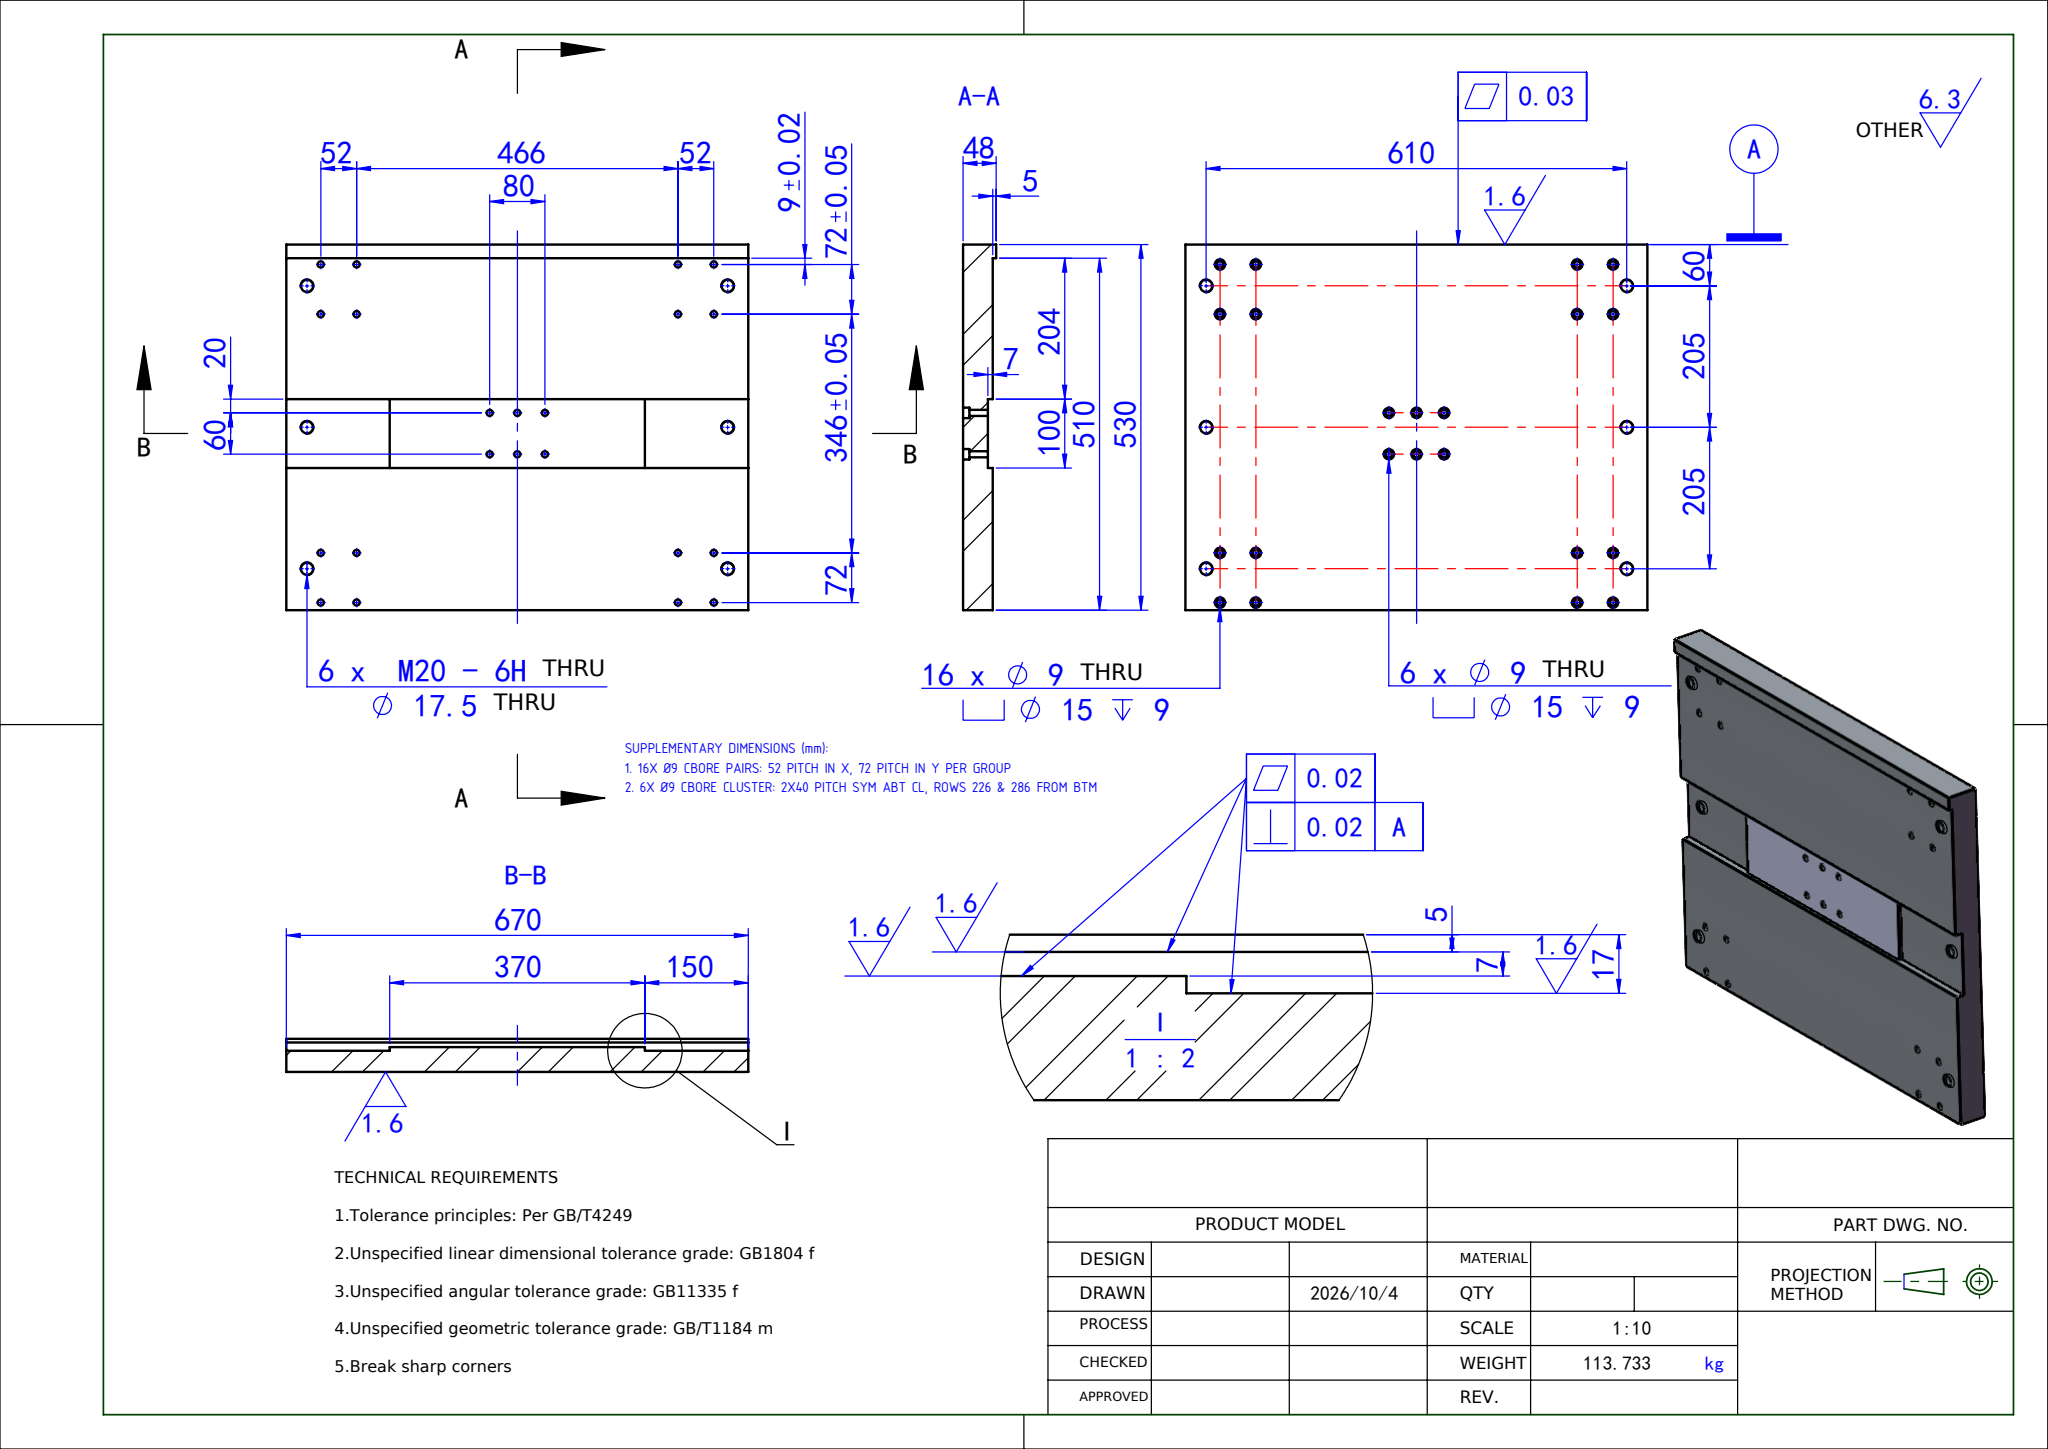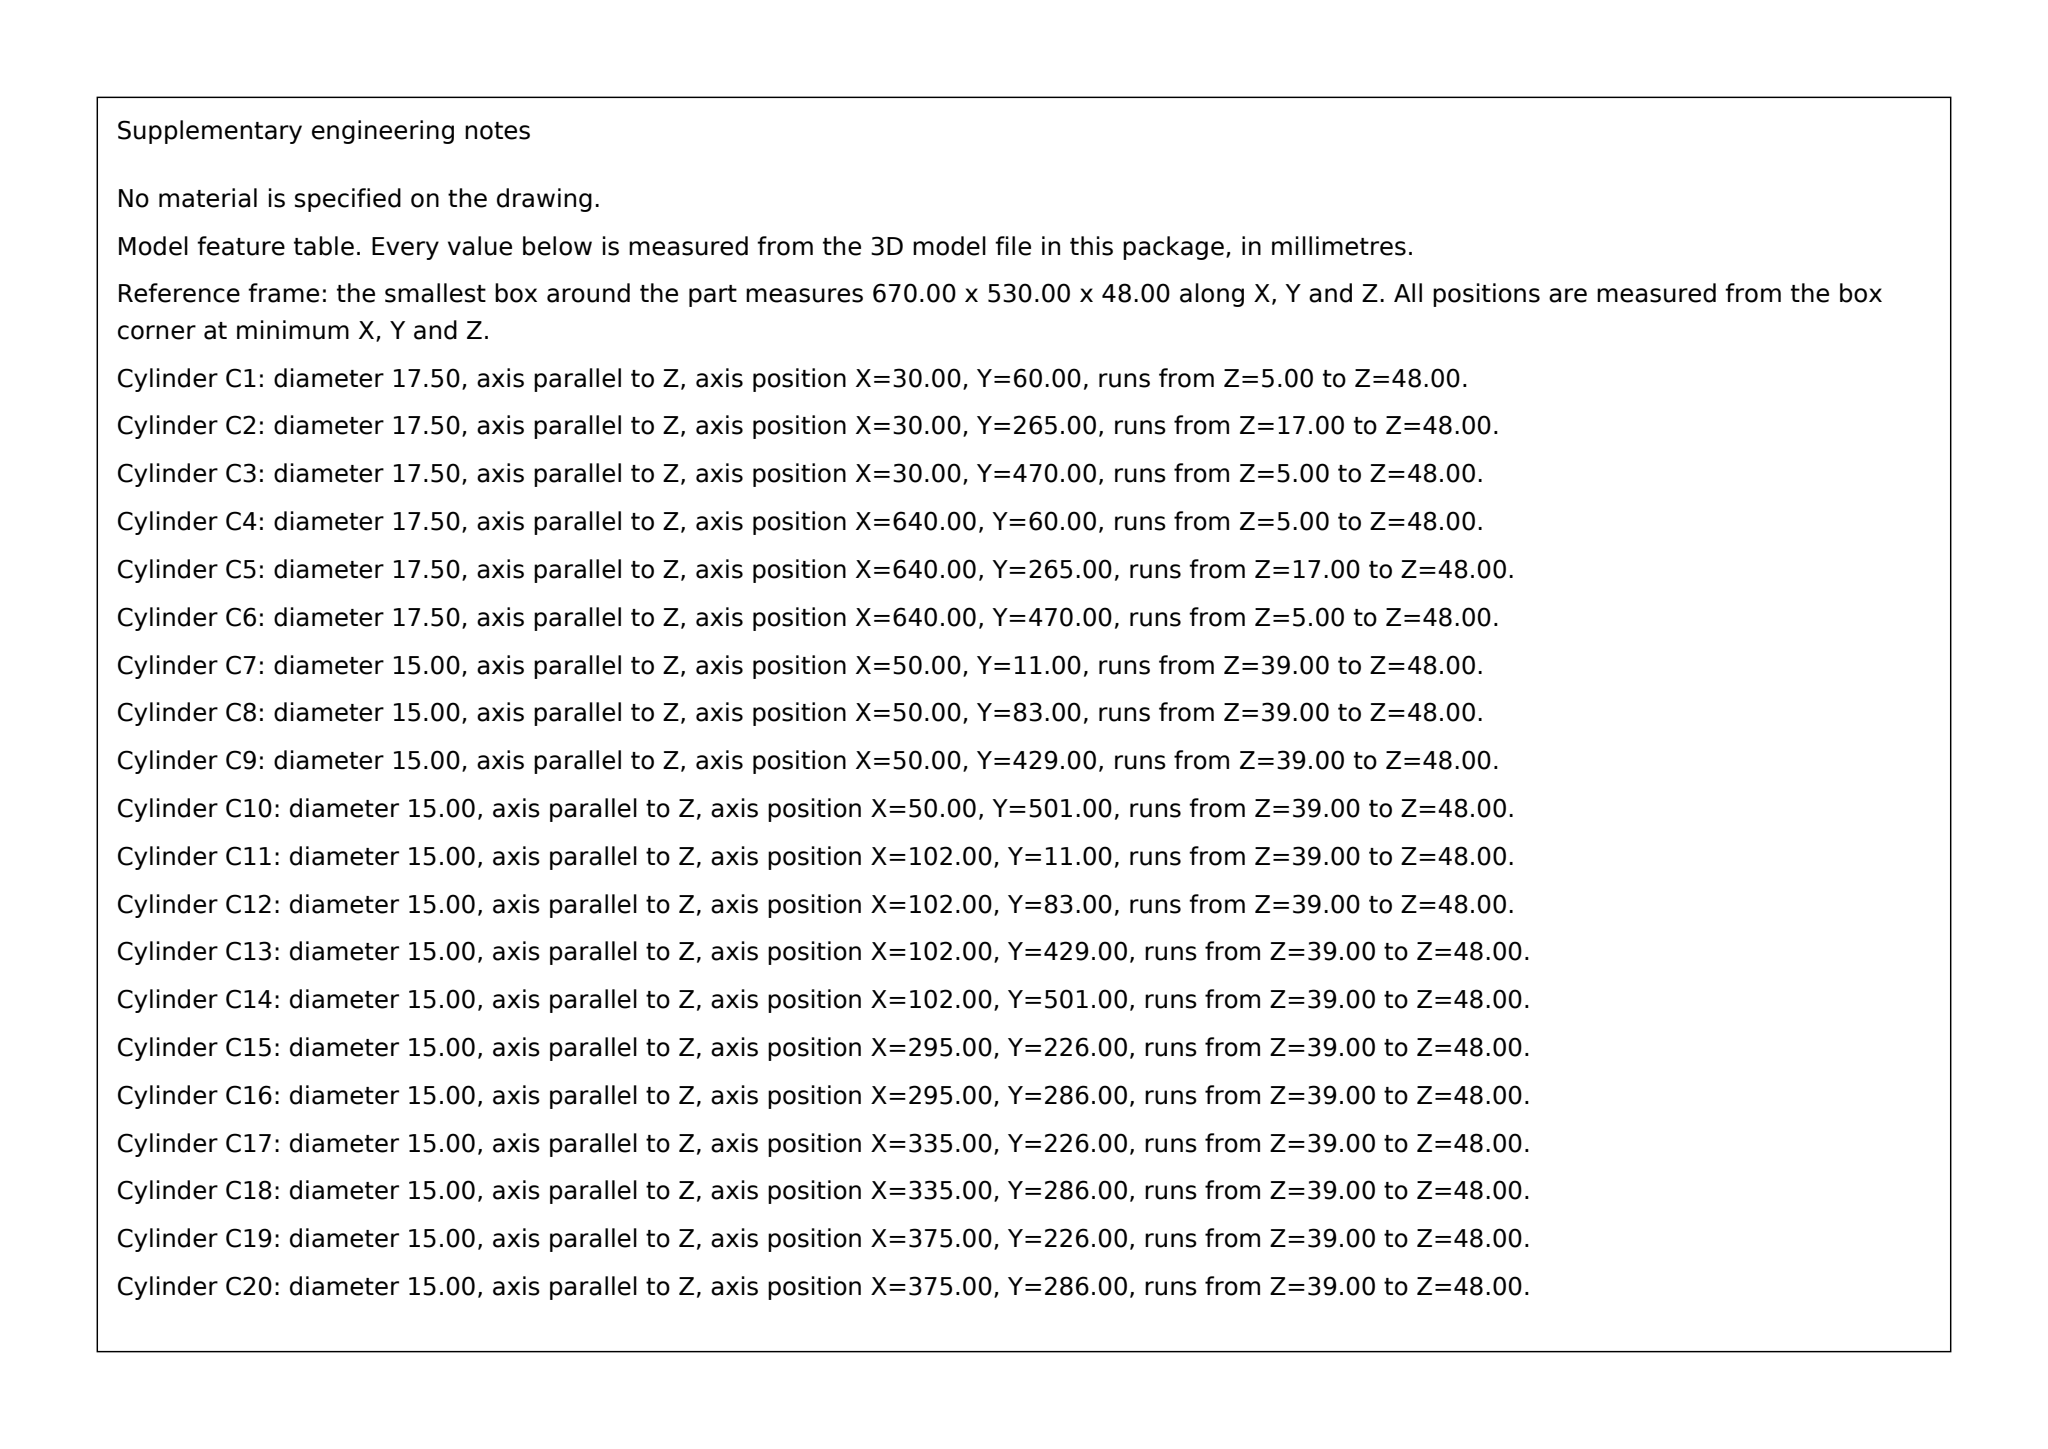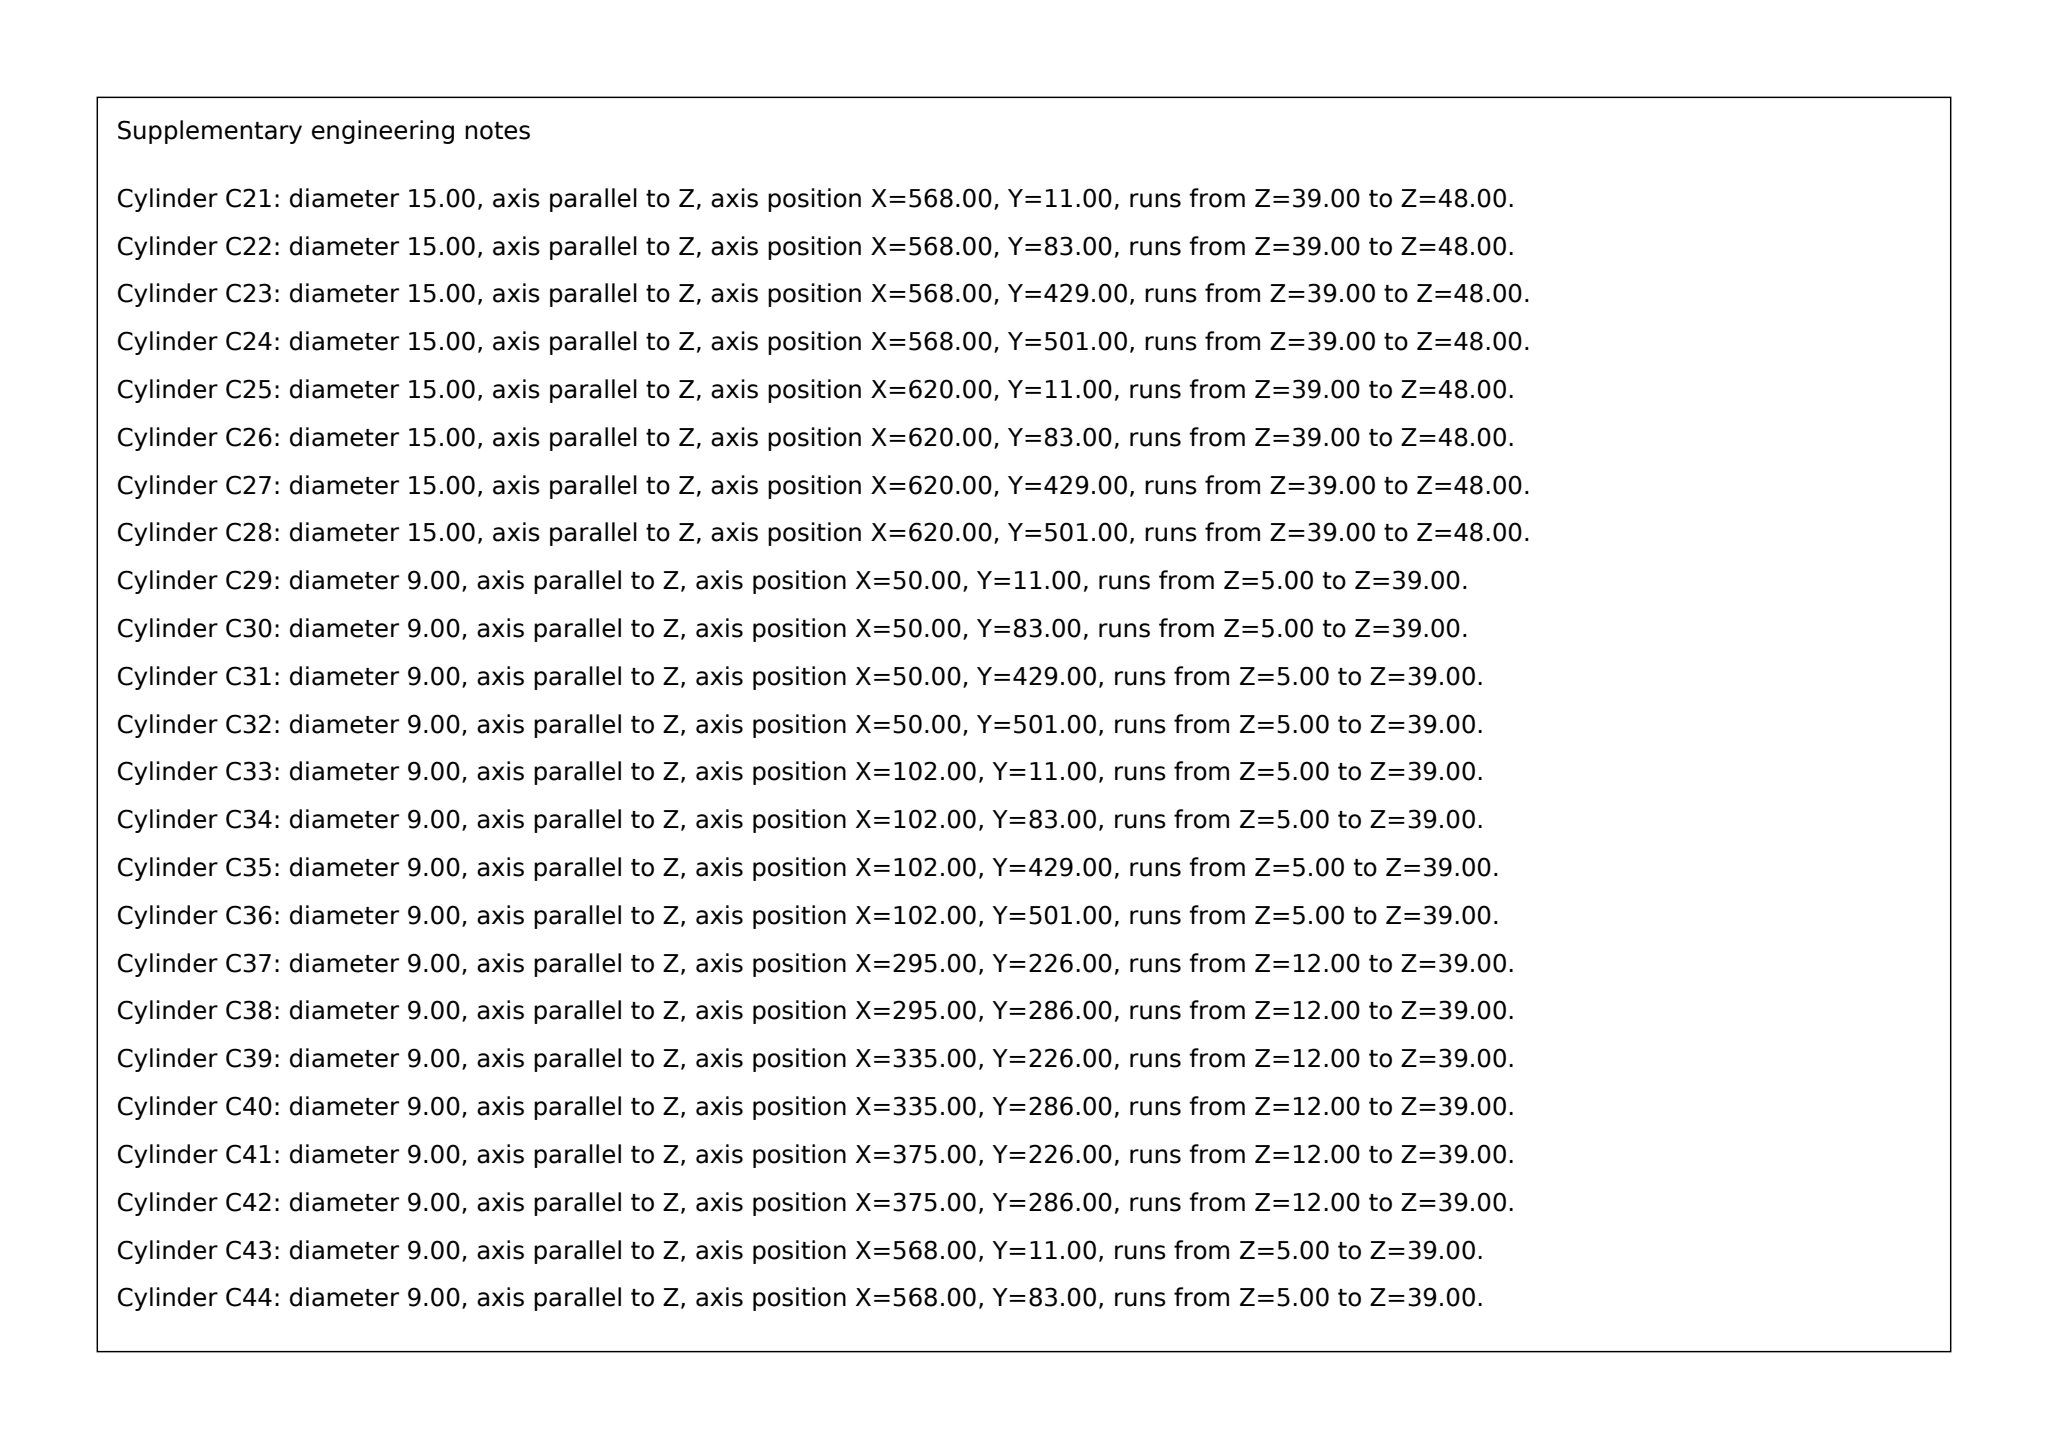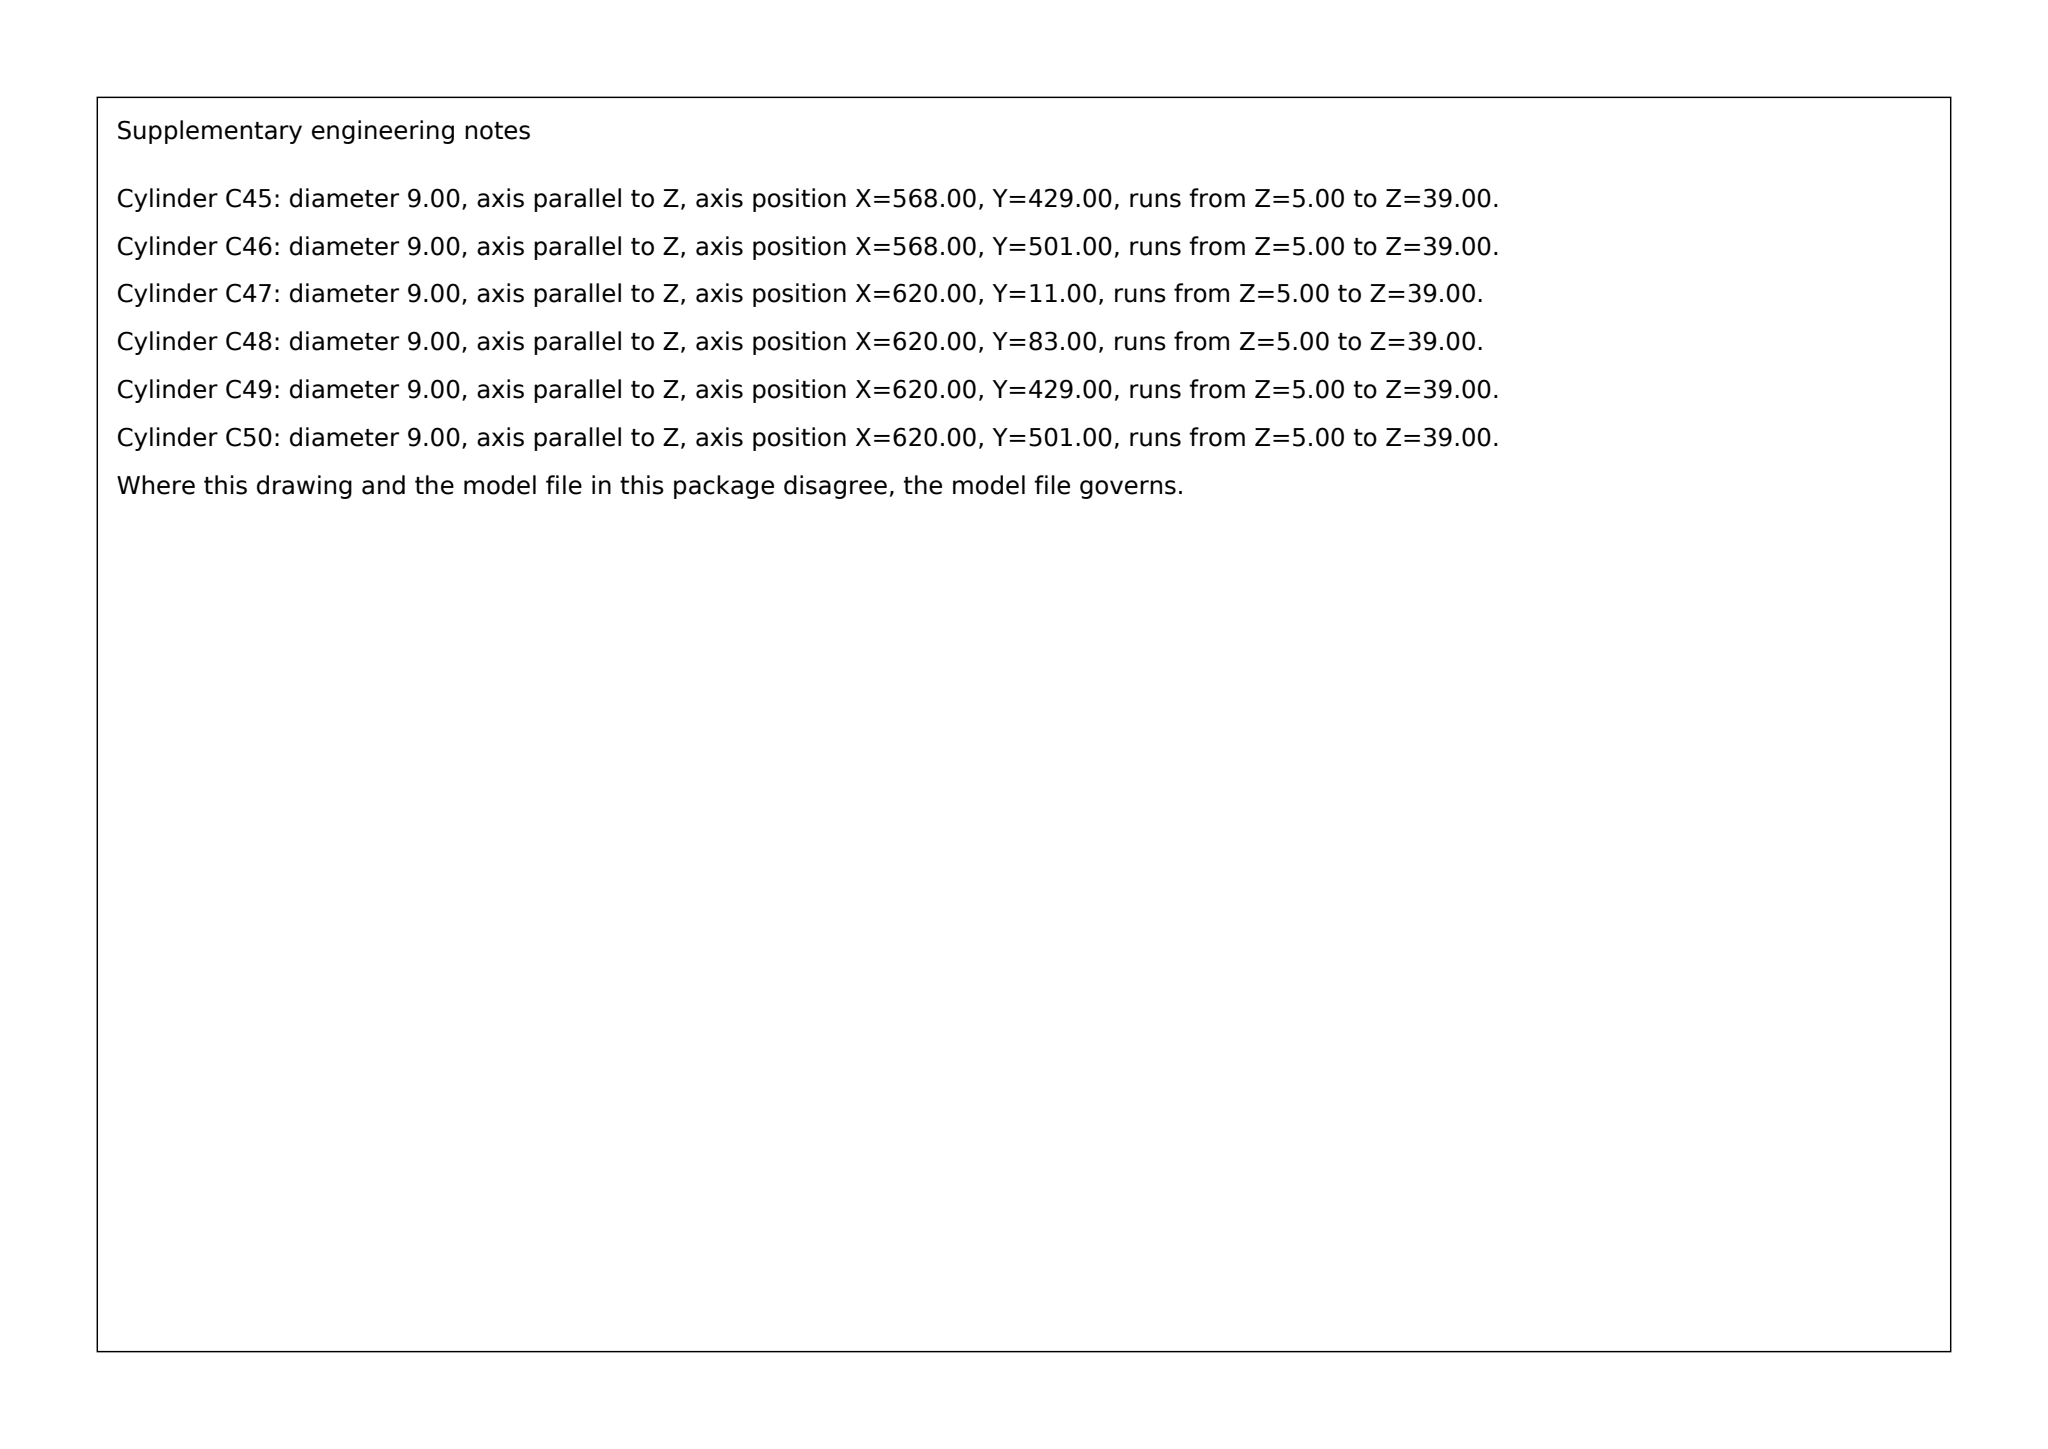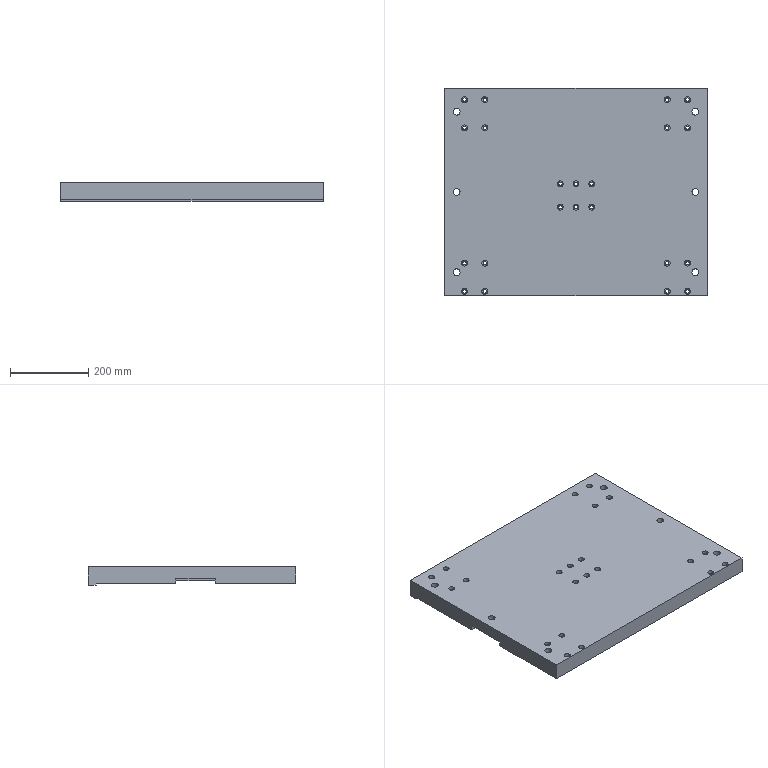Part | SolidWorks | mm | 1 solid | 138 faces | box 670 x 530 x 48 mm | volume 14581113 mm3 | cylinder 100 | plane 38 | commonest cylinder face diameters 15 x44 9 x44 17.5 x12
build123d program:
from build123d import *

# Parameters (mm, degrees)
SKETCH1_W                                         = 670
SKETCH1_H                                         = 530
BOSS_EXTRUDE1_DEPTH                               = 48
M20_TAPPED_HOLE1_D                                = 17.5
SKETCH11_W                                        = 670
SKETCH11_H                                        = 510
CUT_EXTRUDE1_DEPTH                                = 5
HOLE_SIZE_ACCORDING_TO_HEXAGON_SOCKET_D           = 9
HOLE_SIZE_ACCORDING_TO_HEXAGON_SOCKET_CBORE_D     = 15
HOLE_SIZE_ACCORDING_TO_HEXAGON_SOCKET_CBORE_DEPTH = 9
SKETCH14_W                                        = 670
SKETCH14_H                                        = 100
CUT_EXTRUDE2_DEPTH                                = 7
HOLE_SIZE_ACCORDING_TO_HEXAGON_SO_2_D             = 9
HOLE_SIZE_ACCORDING_TO_HEXAGON_SO_2_CBORE_D       = 15
HOLE_SIZE_ACCORDING_TO_HEXAGON_SO_2_CBORE_DEPTH   = 9
SKETCH17_W                                        = 150
SKETCH17_H                                        = 100
CUT_EXTRUDE3_DEPTH                                = 5


with BuildPart() as part:
    # Sketch1 → Boss-Extrude1 (new body)
    with BuildSketch(Plane.XY):
        Rectangle(SKETCH1_W, SKETCH1_H)
    extrude(amount=-BOSS_EXTRUDE1_DEPTH)

    # M20 Tapped Hole1 (through all)
    with Locations(Plane(origin=(0, 0, -48), x_dir=(-1, 0, 0), z_dir=(0, 0, -1))):
        with Locations((-305, 205), (-305, 0), (-305, -205), (305, -205), (305, 0), (305, 205)):
            Hole(M20_TAPPED_HOLE1_D / 2)

    # Sketch11 → Cut-Extrude1 (cut)
    with BuildSketch(Plane(origin=(0, 0, -48), x_dir=(-1, 0, 0), z_dir=(0, 0, -1))):
        with Locations((0, -10)):
            Rectangle(SKETCH11_W, SKETCH11_H)
    extrude(amount=-CUT_EXTRUDE1_DEPTH, mode=Mode.SUBTRACT)

    # Hole Size _ according to_ Hexagon Socket (through all)
    with Locations(Plane.XY):
        with Locations((-285, 236), (-233, 236), (-285, 164), (-233, 164), (-285, -182), (-233, -182), (-233, -254), (-285, -254), (285, -254), (233, -254), (233, -182), (285, -182), (233, 164), (285, 164), (233, 236), (285, 236)):
            CounterBoreHole(HOLE_SIZE_ACCORDING_TO_HEXAGON_SOCKET_D / 2, HOLE_SIZE_ACCORDING_TO_HEXAGON_SOCKET_CBORE_D / 2, HOLE_SIZE_ACCORDING_TO_HEXAGON_SOCKET_CBORE_DEPTH)

    # Sketch14 → Cut-Extrude2 (cut)
    with BuildSketch(Plane(origin=(0, 0, -43), x_dir=(-1, 0, 0), z_dir=(0, 0, -1))):
        with Locations((0, -9)):
            Rectangle(SKETCH14_W, SKETCH14_H)
    extrude(amount=-CUT_EXTRUDE2_DEPTH, mode=Mode.SUBTRACT)

    # Hole Size _ according to_ Hexagon So 2 (through all)
    with Locations(Plane.XY):
        with Locations((-40, 21), (0, 21), (40, 21), (40, -39), (0, -39), (-40, -39)):
            CounterBoreHole(HOLE_SIZE_ACCORDING_TO_HEXAGON_SO_2_D / 2, HOLE_SIZE_ACCORDING_TO_HEXAGON_SO_2_CBORE_D / 2, HOLE_SIZE_ACCORDING_TO_HEXAGON_SO_2_CBORE_DEPTH)

    # Sketch17 → Cut-Extrude3 (cut)
    with BuildSketch(Plane(origin=(0, 0, -36), x_dir=(-1, 0, 0), z_dir=(0, 0, -1))):
        with Locations((-260, -9)):
            Rectangle(SKETCH17_W, SKETCH17_H)
        with Locations((260, -9)):
            Rectangle(SKETCH17_W, SKETCH17_H)
    extrude(amount=-CUT_EXTRUDE3_DEPTH, mode=Mode.SUBTRACT)


solid = part.part